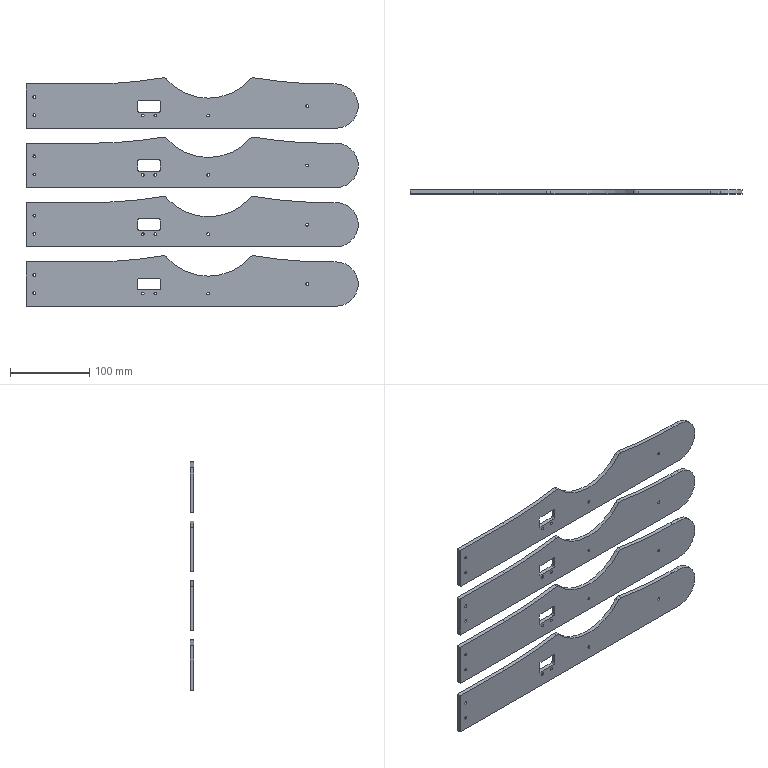CAM job | Mastercam | mm | 4 operations | part box 420 x 5 x 288.8
1. Contour (Ramp) | 3 - 3 平铣刀
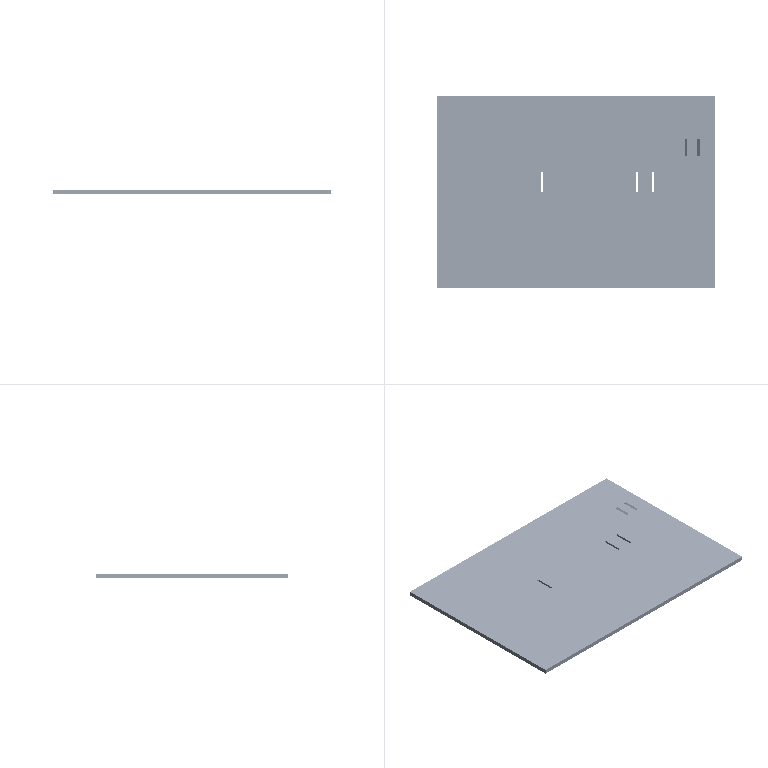2. Contour (2D) | 3 - 3 平铣刀
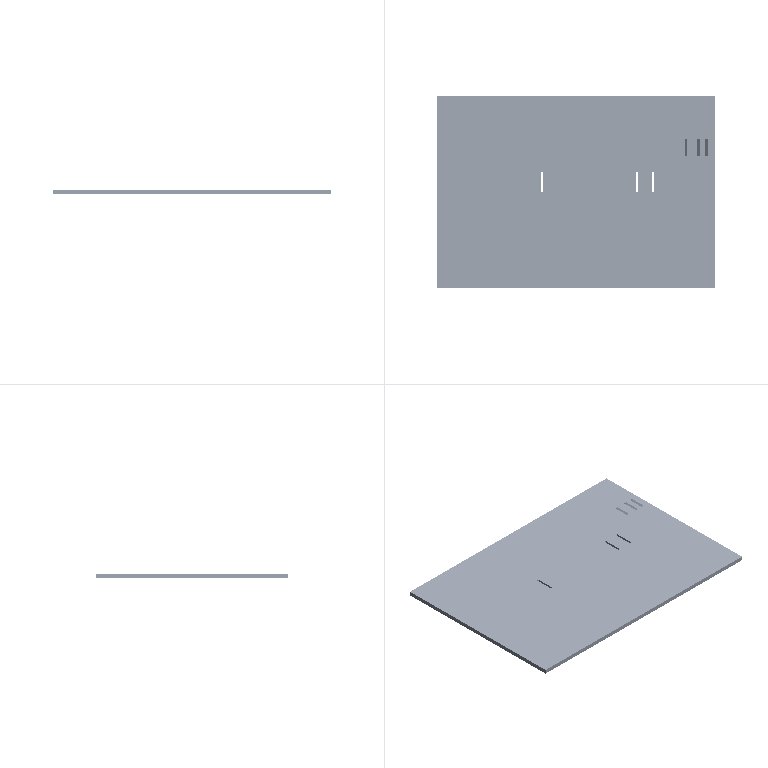3. Drill/Counterbore | 7 - 4 倒角刀
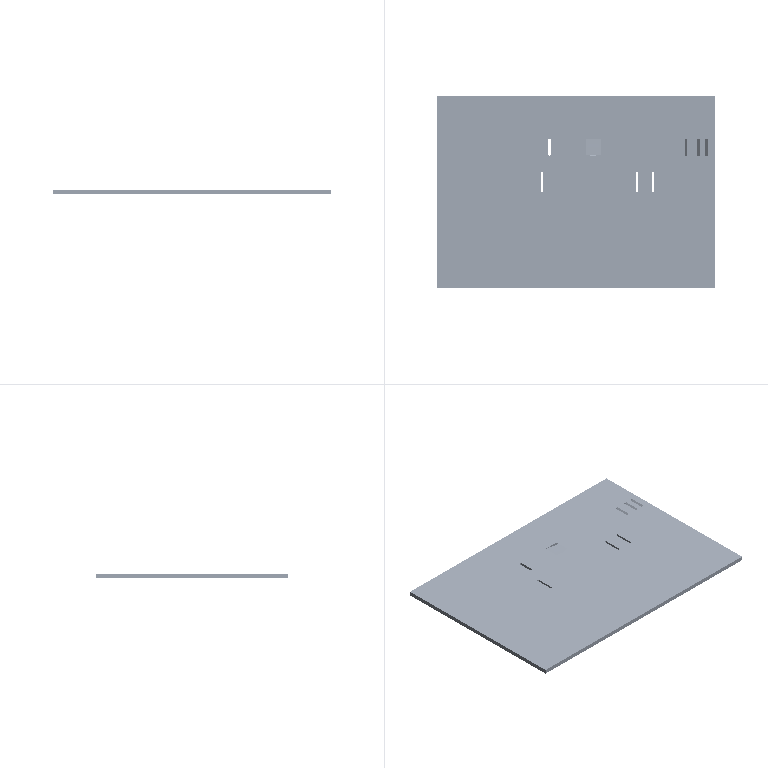4. Contour (2D chamfer) | 7 - 4 倒角刀